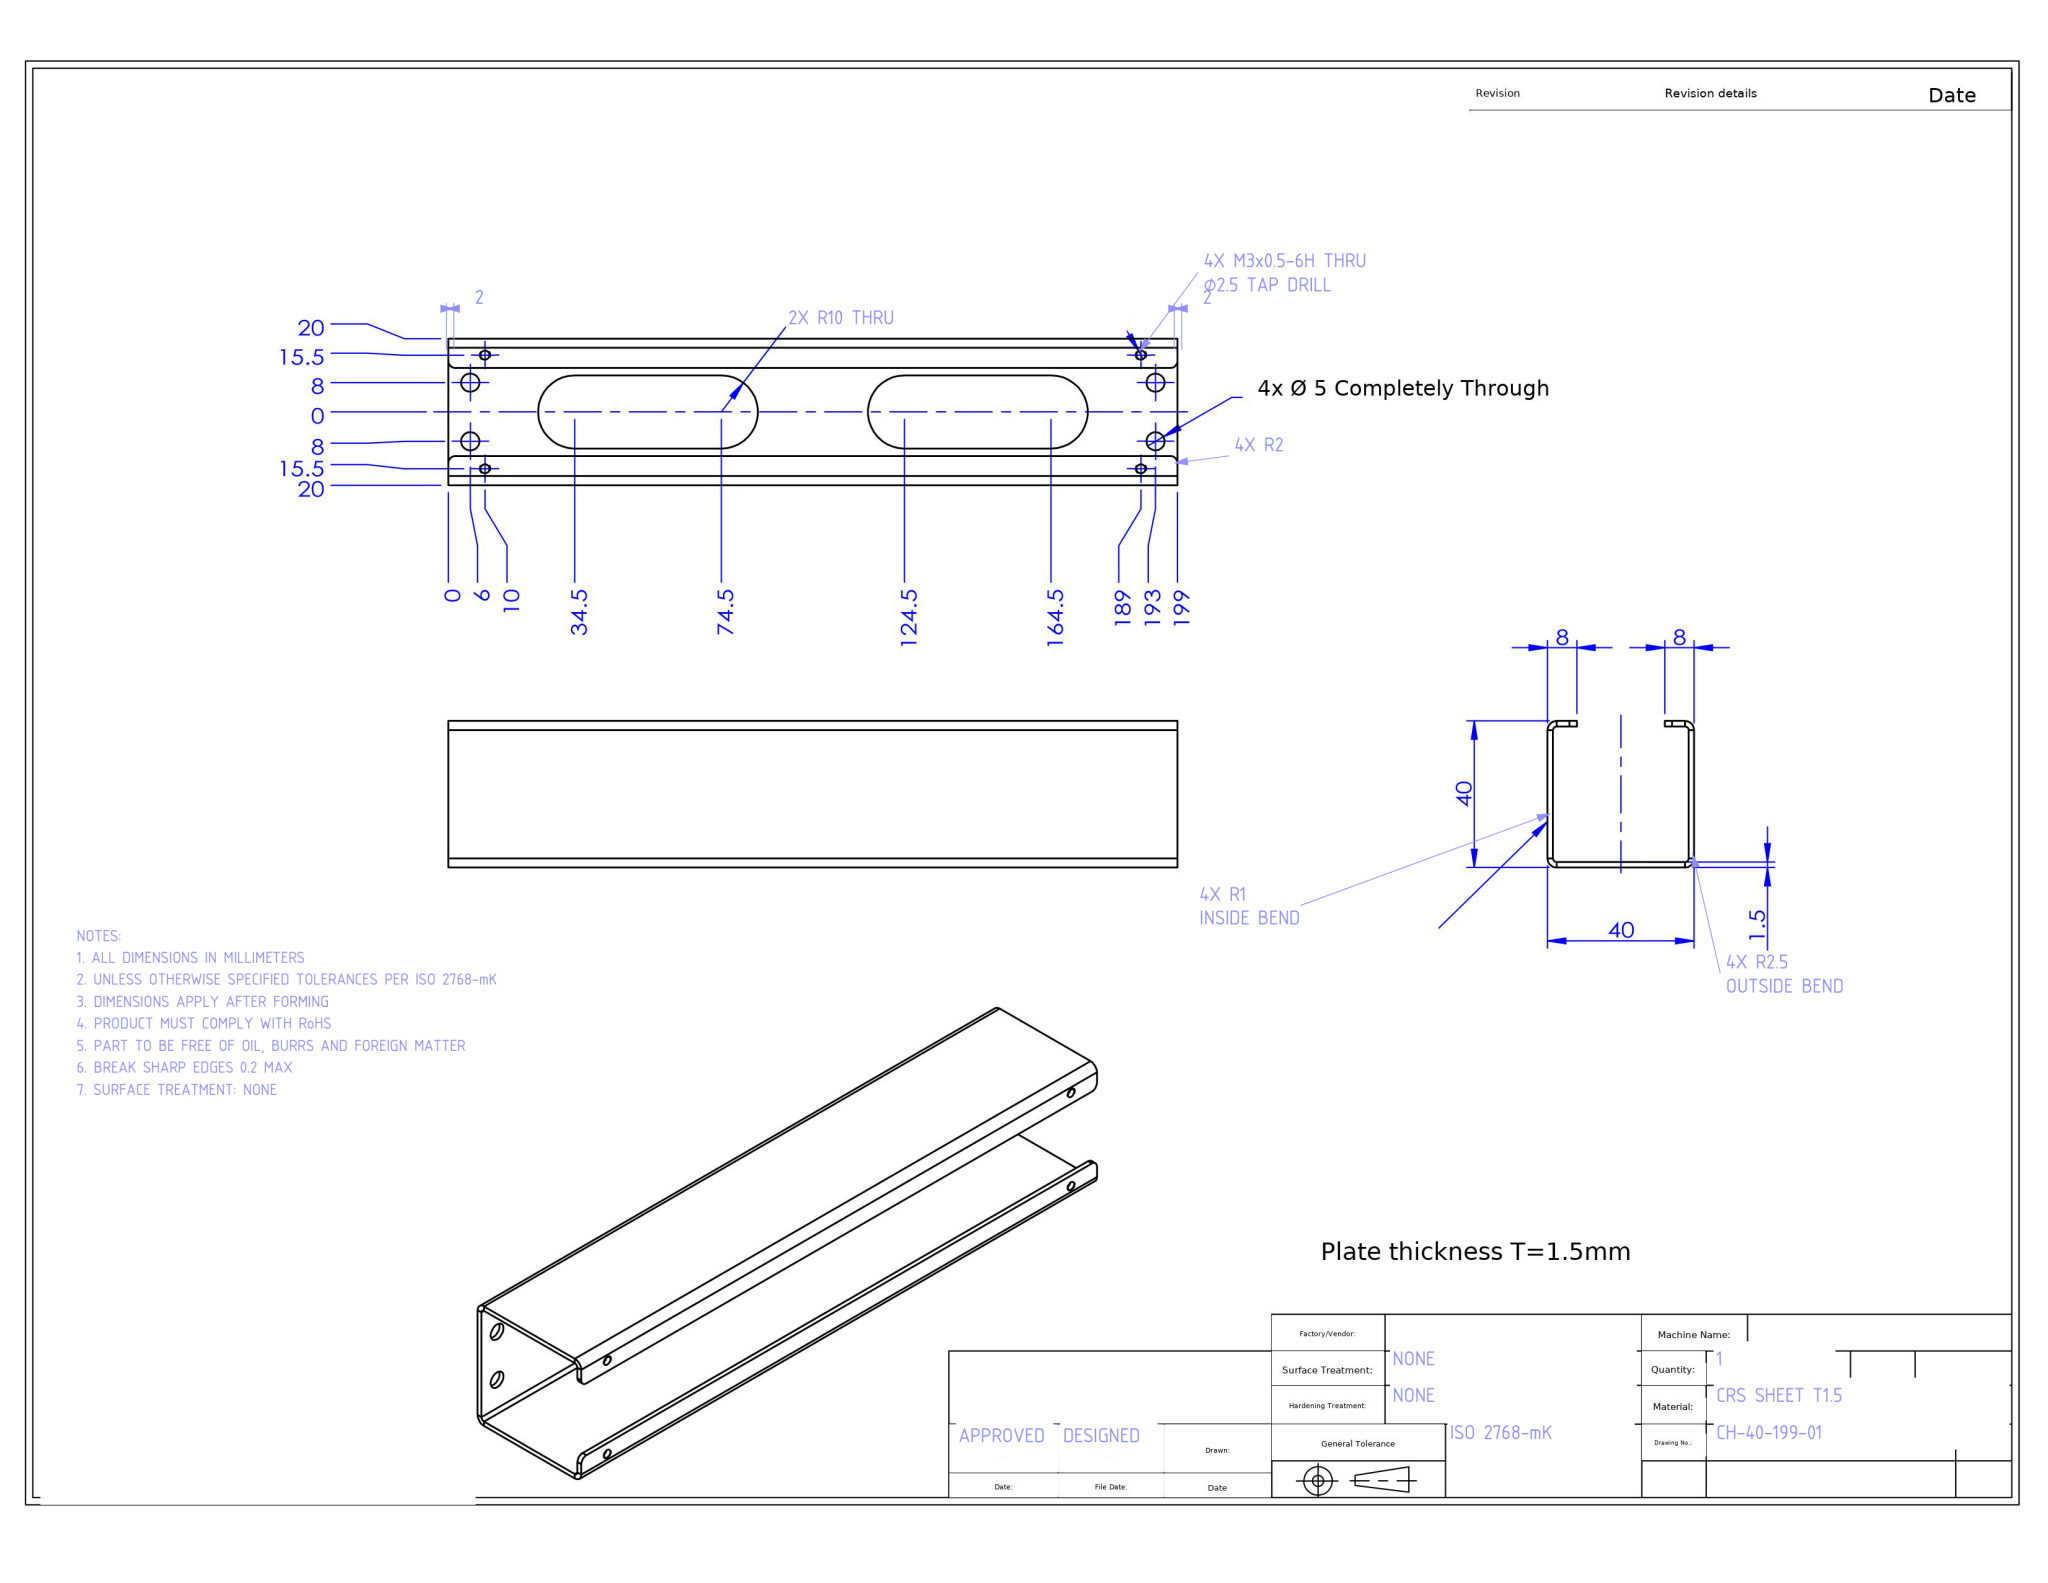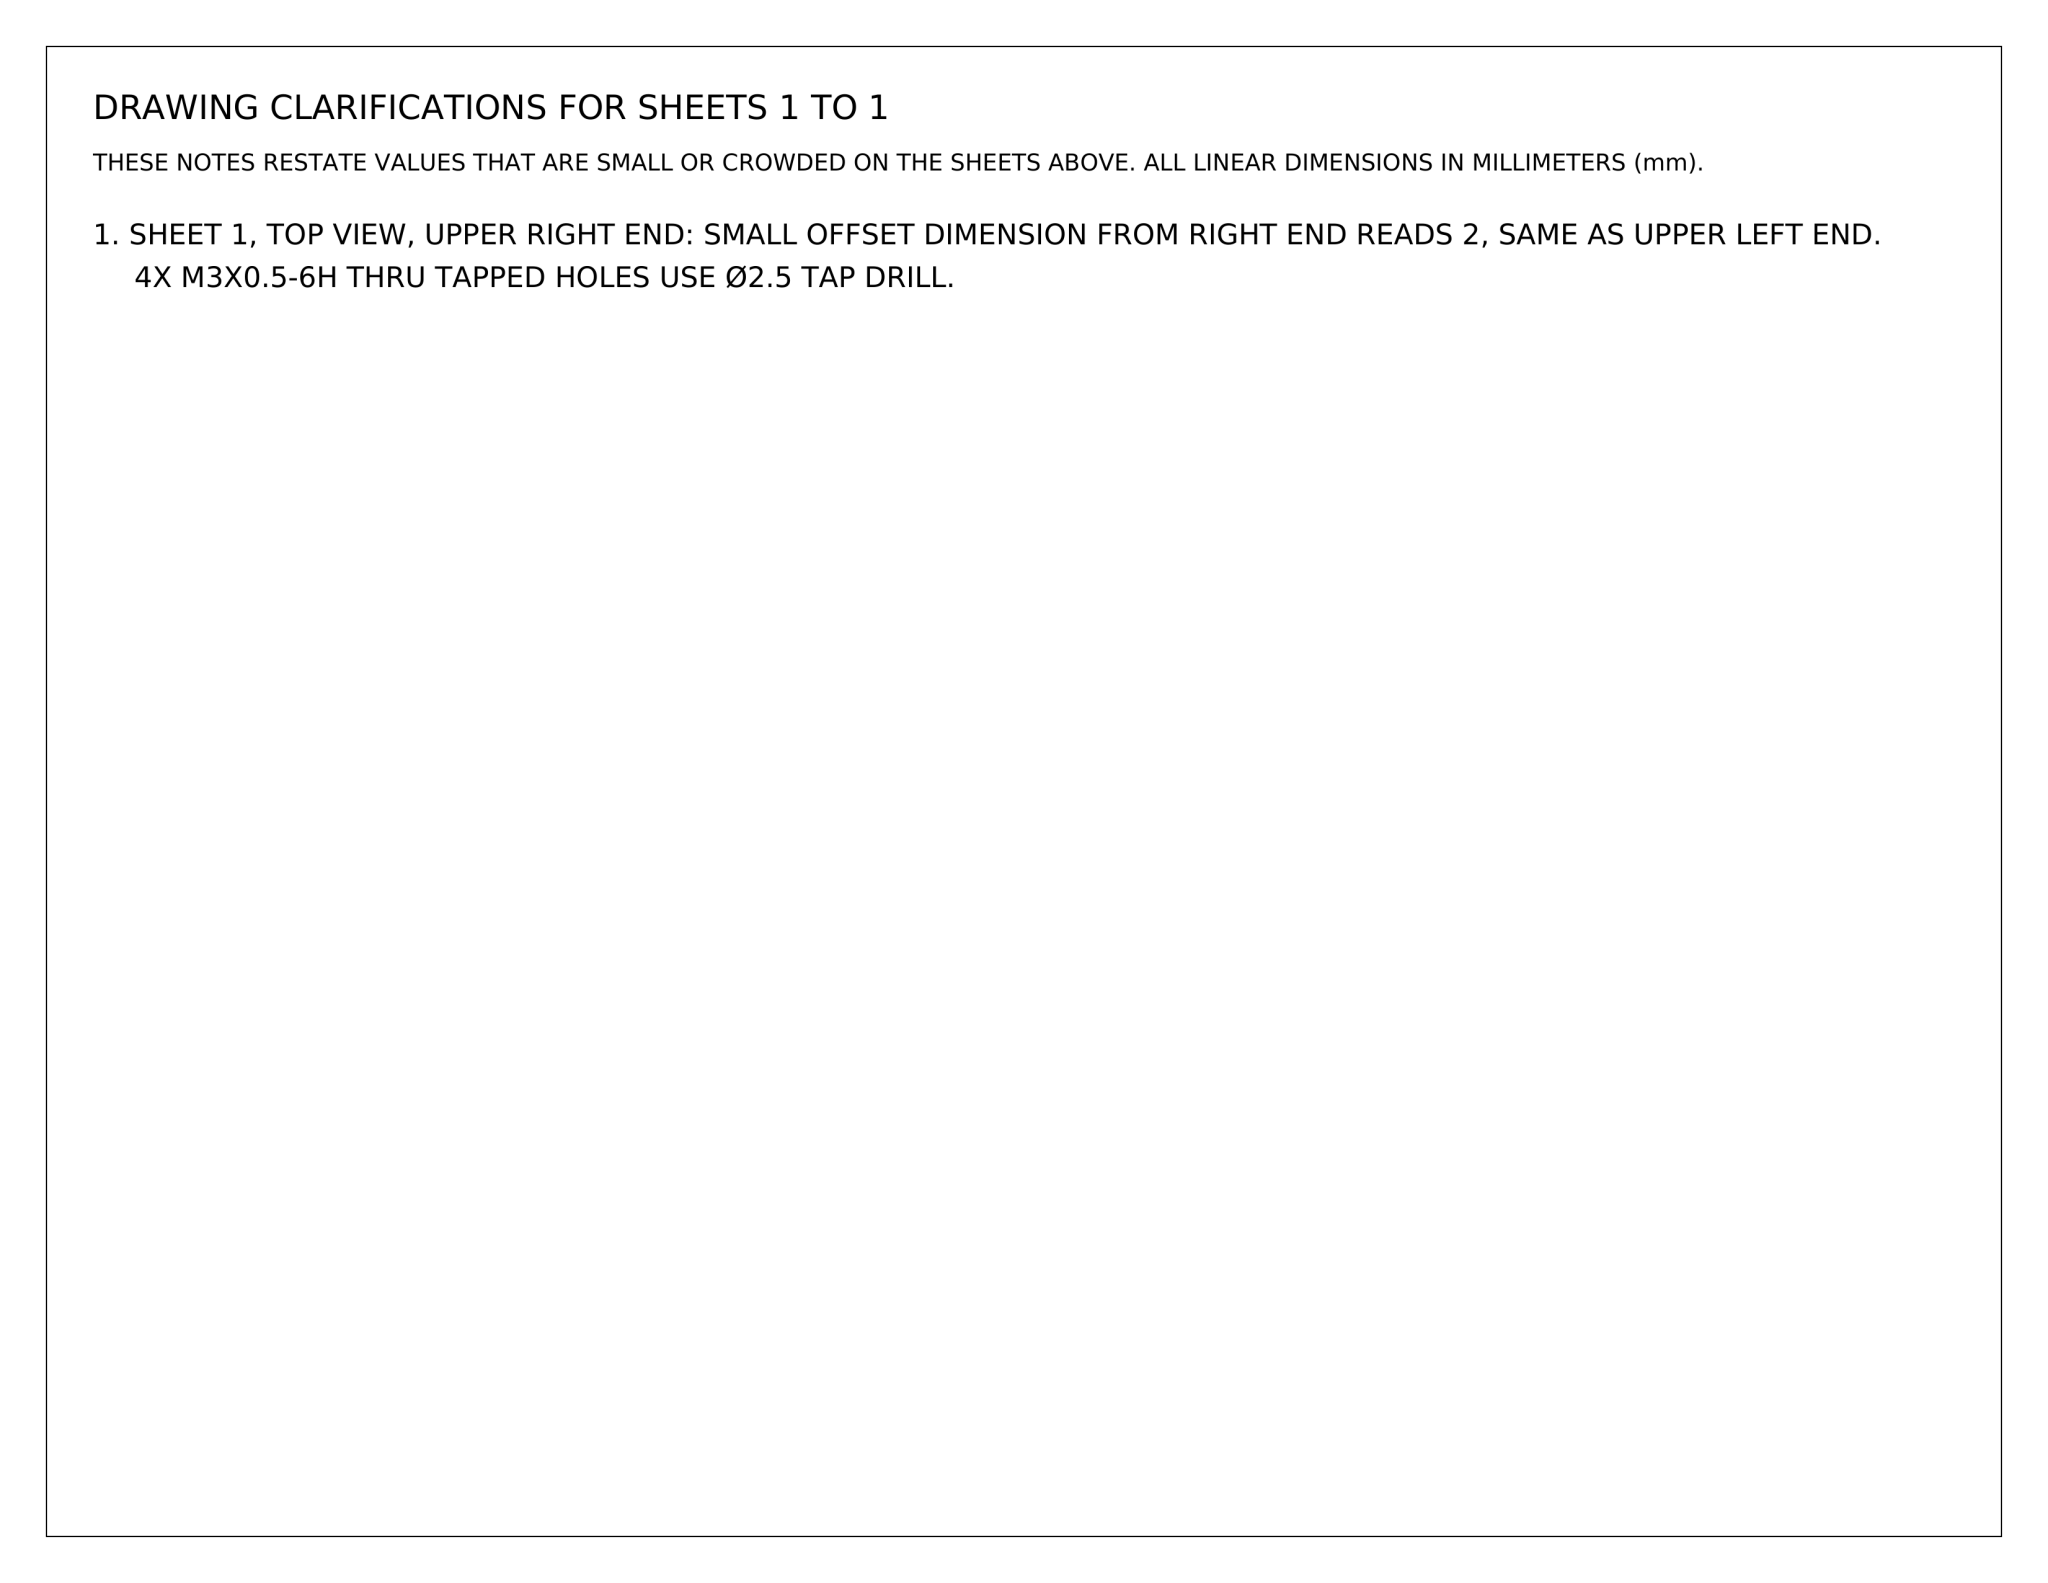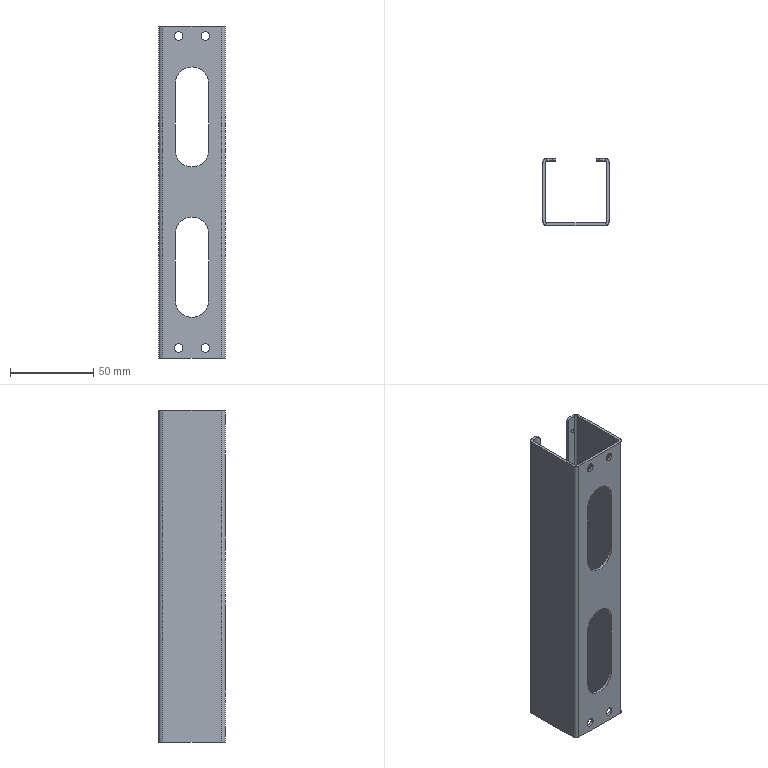Part | NX | mm | 1 solid | 68 faces | box 40 x 40 x 199 mm | volume 34413 mm3 | cylinder 34 | plane 34 | commonest cylinder face diameters 5 x12 2.5 x8 20 x6 2 x4 4 x4